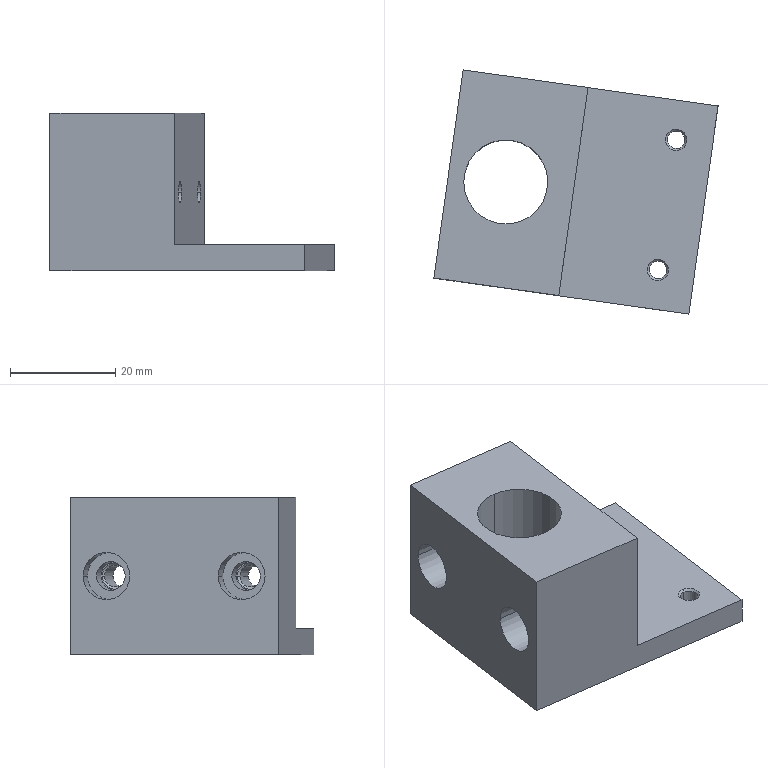Component | SolidWorks | SwitchMount-1 | 1 solid | 38 faces | box 54.1 x 46.44 x 30 mm | volume 26297 mm3 | cylinder 18 | plane 12 | cone 8 | commonest cylinder face diameters 3.3 x4 5.5 x4 4.2 x4 9 x4 16 x2
STEP:
#1=CARTESIAN_POINT('',(-2.788,-8.94,0.7923));
#2=VERTEX_POINT('',#1);
#3=CARTESIAN_POINT('',(-2.806,-9.068,0.7923));
#4=VERTEX_POINT('',#3);
#5=CARTESIAN_POINT('',(-2.797,-9.004,0.7923));
#6=DIRECTION('',(-0.,0.,1.));
#7=DIRECTION('',(-0.1393,-0.9902,0.));
#8=AXIS2_PLACEMENT_3D('',#5,#6,#7);
#9=CIRCLE('',#8,0.06496);
#10=EDGE_CURVE('',#2,#4,#9,.T.);
#11=ORIENTED_EDGE('',*,*,#10,.F.);
#12=CARTESIAN_POINT('',(-2.786,-8.925,0.8071));
#13=VERTEX_POINT('',#12);
#14=CARTESIAN_POINT('',(-2.786,-8.925,0.8071));
#15=DIRECTION('',(0.09852,0.7002,0.7071));
#16=VECTOR('',#15,39.37);
#17=LINE('',#14,#16);
#18=EDGE_CURVE('',#2,#13,#17,.T.);
#19=ORIENTED_EDGE('',*,*,#18,.T.);
#20=CARTESIAN_POINT('',(-2.808,-9.083,0.8071));
#21=VERTEX_POINT('',#20);
#22=CARTESIAN_POINT('',(-2.797,-9.004,0.8071));
#23=DIRECTION('',(-0.,0.,1.));
#24=DIRECTION('',(-0.1393,-0.9902,0.));
#25=AXIS2_PLACEMENT_3D('',#22,#23,#24);
#26=CIRCLE('',#25,0.07972);
#27=EDGE_CURVE('',#13,#21,#26,.T.);
#28=ORIENTED_EDGE('',*,*,#27,.T.);
#29=CARTESIAN_POINT('',(-2.808,-9.083,0.8071));
#30=DIRECTION('',(-0.09852,-0.7002,0.7071));
#31=VECTOR('',#30,39.37);
#32=LINE('',#29,#31);
#33=EDGE_CURVE('',#4,#21,#32,.T.);
#34=ORIENTED_EDGE('',*,*,#33,.F.);
#35=EDGE_LOOP('',(#11,#19,#28,#34));
#36=FACE_OUTER_BOUND('',#35,.T.);
#37=CARTESIAN_POINT('',(-2.797,-9.004,0.8071));
#38=DIRECTION('',(-0.,0.,1.));
#39=DIRECTION('',(-0.1393,-0.9902,0.));
#40=AXIS2_PLACEMENT_3D('',#37,#38,#39);
#41=CONICAL_SURFACE('',#40,0.07972,0.7854);
#42=ADVANCED_FACE('',(#36),#41,.F.);
#43=CARTESIAN_POINT('',(-2.788,-8.94,0.6102));
#44=VERTEX_POINT('',#43);
#45=CARTESIAN_POINT('',(-2.806,-9.068,0.6102));
#46=VERTEX_POINT('',#45);
#47=CARTESIAN_POINT('',(-2.797,-9.004,0.6102));
#48=DIRECTION('',(-0.,0.,1.));
#49=DIRECTION('',(-0.1393,-0.9902,0.));
#50=AXIS2_PLACEMENT_3D('',#47,#48,#49);
#51=CIRCLE('',#50,0.06496);
#52=EDGE_CURVE('',#44,#46,#51,.T.);
#53=ORIENTED_EDGE('',*,*,#52,.F.);
#54=CARTESIAN_POINT('',(-2.788,-8.94,0.8071));
#55=DIRECTION('',(-0.,0.,1.));
#56=VECTOR('',#55,39.37);
#57=LINE('',#54,#56);
#58=EDGE_CURVE('',#44,#2,#57,.T.);
#59=ORIENTED_EDGE('',*,*,#58,.T.);
#60=ORIENTED_EDGE('',*,*,#10,.T.);
#61=CARTESIAN_POINT('',(-2.806,-9.068,0.8071));
#62=DIRECTION('',(-0.,0.,1.));
#63=VECTOR('',#62,39.37);
#64=LINE('',#61,#63);
#65=EDGE_CURVE('',#46,#4,#64,.T.);
#66=ORIENTED_EDGE('',*,*,#65,.F.);
#67=EDGE_LOOP('',(#53,#59,#60,#66));
#68=FACE_OUTER_BOUND('',#67,.T.);
#69=CARTESIAN_POINT('',(-2.797,-9.004,0.8071));
#70=DIRECTION('',(-0.,0.,1.));
#71=DIRECTION('',(-0.1393,-0.9902,0.));
#72=AXIS2_PLACEMENT_3D('',#69,#70,#71);
#73=CYLINDRICAL_SURFACE('',#72,0.06496);
#74=ADVANCED_FACE('',(#68),#73,.F.);
#75=CARTESIAN_POINT('',(-2.651,-7.965,0.7923));
#76=VERTEX_POINT('',#75);
#77=CARTESIAN_POINT('',(-2.669,-8.094,0.7923));
#78=VERTEX_POINT('',#77);
#79=CARTESIAN_POINT('',(-2.66,-8.029,0.7923));
#80=DIRECTION('',(-0.,0.,1.));
#81=DIRECTION('',(-0.1393,-0.9902,0.));
#82=AXIS2_PLACEMENT_3D('',#79,#80,#81);
#83=CIRCLE('',#82,0.06496);
#84=EDGE_CURVE('',#76,#78,#83,.T.);
#85=ORIENTED_EDGE('',*,*,#84,.F.);
#86=CARTESIAN_POINT('',(-2.649,-7.95,0.8071));
#87=VERTEX_POINT('',#86);
#88=CARTESIAN_POINT('',(-2.649,-7.95,0.8071));
#89=DIRECTION('',(0.09852,0.7002,0.7071));
#90=VECTOR('',#89,39.37);
#91=LINE('',#88,#90);
#92=EDGE_CURVE('',#76,#87,#91,.T.);
#93=ORIENTED_EDGE('',*,*,#92,.T.);
#94=CARTESIAN_POINT('',(-2.671,-8.108,0.8071));
#95=VERTEX_POINT('',#94);
#96=CARTESIAN_POINT('',(-2.66,-8.029,0.8071));
#97=DIRECTION('',(-0.,0.,1.));
#98=DIRECTION('',(-0.1393,-0.9902,0.));
#99=AXIS2_PLACEMENT_3D('',#96,#97,#98);
#100=CIRCLE('',#99,0.07972);
#101=EDGE_CURVE('',#87,#95,#100,.T.);
#102=ORIENTED_EDGE('',*,*,#101,.T.);
#103=CARTESIAN_POINT('',(-2.671,-8.108,0.8071));
#104=DIRECTION('',(-0.09852,-0.7002,0.7071));
#105=VECTOR('',#104,39.37);
#106=LINE('',#103,#105);
#107=EDGE_CURVE('',#78,#95,#106,.T.);
#108=ORIENTED_EDGE('',*,*,#107,.F.);
#109=EDGE_LOOP('',(#85,#93,#102,#108));
#110=FACE_OUTER_BOUND('',#109,.T.);
#111=CARTESIAN_POINT('',(-2.66,-8.029,0.8071));
#112=DIRECTION('',(-0.,0.,1.));
#113=DIRECTION('',(-0.1393,-0.9902,0.));
#114=AXIS2_PLACEMENT_3D('',#111,#112,#113);
#115=CONICAL_SURFACE('',#114,0.07972,0.7854);
#116=ADVANCED_FACE('',(#110),#115,.F.);
#117=CARTESIAN_POINT('',(-2.651,-7.965,0.6102));
#118=VERTEX_POINT('',#117);
#119=CARTESIAN_POINT('',(-2.669,-8.094,0.6102));
#120=VERTEX_POINT('',#119);
#121=CARTESIAN_POINT('',(-2.66,-8.029,0.6102));
#122=DIRECTION('',(-0.,0.,1.));
#123=DIRECTION('',(-0.1393,-0.9902,0.));
#124=AXIS2_PLACEMENT_3D('',#121,#122,#123);
#125=CIRCLE('',#124,0.06496);
#126=EDGE_CURVE('',#118,#120,#125,.T.);
#127=ORIENTED_EDGE('',*,*,#126,.F.);
#128=CARTESIAN_POINT('',(-2.651,-7.965,0.8071));
#129=DIRECTION('',(-0.,0.,1.));
#130=VECTOR('',#129,39.37);
#131=LINE('',#128,#130);
#132=EDGE_CURVE('',#118,#76,#131,.T.);
#133=ORIENTED_EDGE('',*,*,#132,.T.);
#134=ORIENTED_EDGE('',*,*,#84,.T.);
#135=CARTESIAN_POINT('',(-2.669,-8.094,0.8071));
#136=DIRECTION('',(-0.,0.,1.));
#137=VECTOR('',#136,39.37);
#138=LINE('',#135,#137);
#139=EDGE_CURVE('',#120,#78,#138,.T.);
#140=ORIENTED_EDGE('',*,*,#139,.F.);
#141=EDGE_LOOP('',(#127,#133,#134,#140));
#142=FACE_OUTER_BOUND('',#141,.T.);
#143=CARTESIAN_POINT('',(-2.66,-8.029,0.8071));
#144=DIRECTION('',(-0.,0.,1.));
#145=DIRECTION('',(-0.1393,-0.9902,0.));
#146=AXIS2_PLACEMENT_3D('',#143,#144,#145);
#147=CYLINDRICAL_SURFACE('',#146,0.06496);
#148=ADVANCED_FACE('',(#142),#147,.F.);
#149=CARTESIAN_POINT('',(-3.981,-8.658,1.791));
#150=VERTEX_POINT('',#149);
#151=CARTESIAN_POINT('',(-3.893,-8.035,1.791));
#152=VERTEX_POINT('',#151);
#153=CARTESIAN_POINT('',(-3.937,-8.346,1.791));
#154=DIRECTION('',(0.,-0.,-1.));
#155=DIRECTION('',(0.1393,0.9902,0.));
#156=AXIS2_PLACEMENT_3D('',#153,#154,#155);
#157=CIRCLE('',#156,0.315);
#158=EDGE_CURVE('',#150,#152,#157,.T.);
#159=ORIENTED_EDGE('',*,*,#158,.F.);
#160=CARTESIAN_POINT('',(-3.981,-8.658,0.6102));
#161=VERTEX_POINT('',#160);
#162=CARTESIAN_POINT('',(-3.981,-8.658,0.6102));
#163=DIRECTION('',(0.,-0.,-1.));
#164=VECTOR('',#163,39.37);
#165=LINE('',#162,#164);
#166=EDGE_CURVE('',#150,#161,#165,.T.);
#167=ORIENTED_EDGE('',*,*,#166,.T.);
#168=CARTESIAN_POINT('',(-3.893,-8.035,0.6102));
#169=VERTEX_POINT('',#168);
#170=CARTESIAN_POINT('',(-3.937,-8.346,0.6102));
#171=DIRECTION('',(0.,-0.,-1.));
#172=DIRECTION('',(0.1393,0.9902,0.));
#173=AXIS2_PLACEMENT_3D('',#170,#171,#172);
#174=CIRCLE('',#173,0.315);
#175=EDGE_CURVE('',#161,#169,#174,.T.);
#176=ORIENTED_EDGE('',*,*,#175,.T.);
#177=CARTESIAN_POINT('',(-3.893,-8.035,0.6102));
#178=DIRECTION('',(0.,-0.,-1.));
#179=VECTOR('',#178,39.37);
#180=LINE('',#177,#179);
#181=EDGE_CURVE('',#152,#169,#180,.T.);
#182=ORIENTED_EDGE('',*,*,#181,.F.);
#183=EDGE_LOOP('',(#159,#167,#176,#182));
#184=FACE_OUTER_BOUND('',#183,.T.);
#185=CARTESIAN_POINT('',(-3.937,-8.346,0.6102));
#186=DIRECTION('',(0.,-0.,-1.));
#187=DIRECTION('',(0.1393,0.9902,0.));
#188=AXIS2_PLACEMENT_3D('',#185,#186,#187);
#189=CYLINDRICAL_SURFACE('',#188,0.315);
#190=ADVANCED_FACE('',(#184),#189,.F.);
#191=CARTESIAN_POINT('',(-4.218,-8.933,1.201));
#192=VERTEX_POINT('',#191);
#193=CARTESIAN_POINT('',(-4.188,-8.719,1.201));
#194=VERTEX_POINT('',#193);
#195=CARTESIAN_POINT('',(-4.203,-8.826,1.201));
#196=DIRECTION('',(0.9902,-0.1393,0.));
#197=DIRECTION('',(0.1393,0.9902,0.));
#198=AXIS2_PLACEMENT_3D('',#195,#196,#197);
#199=CIRCLE('',#198,0.1083);
#200=EDGE_CURVE('',#192,#194,#199,.T.);
#201=ORIENTED_EDGE('',*,*,#200,.F.);
#202=CARTESIAN_POINT('',(-3.984,-8.966,1.201));
#203=VERTEX_POINT('',#202);
#204=CARTESIAN_POINT('',(-4.452,-8.9,1.201));
#205=DIRECTION('',(0.9902,-0.1393,0.));
#206=VECTOR('',#205,39.37);
#207=LINE('',#204,#206);
#208=EDGE_CURVE('',#192,#203,#207,.T.);
#209=ORIENTED_EDGE('',*,*,#208,.T.);
#210=CARTESIAN_POINT('',(-3.954,-8.752,1.201));
#211=VERTEX_POINT('',#210);
#212=CARTESIAN_POINT('',(-3.969,-8.859,1.201));
#213=DIRECTION('',(0.9902,-0.1393,0.));
#214=DIRECTION('',(0.1393,0.9902,0.));
#215=AXIS2_PLACEMENT_3D('',#212,#213,#214);
#216=CIRCLE('',#215,0.1083);
#217=EDGE_CURVE('',#203,#211,#216,.T.);
#218=ORIENTED_EDGE('',*,*,#217,.T.);
#219=CARTESIAN_POINT('',(-4.422,-8.686,1.201));
#220=DIRECTION('',(0.9902,-0.1393,0.));
#221=VECTOR('',#220,39.37);
#222=LINE('',#219,#221);
#223=EDGE_CURVE('',#194,#211,#222,.T.);
#224=ORIENTED_EDGE('',*,*,#223,.F.);
#225=EDGE_LOOP('',(#201,#209,#218,#224));
#226=FACE_OUTER_BOUND('',#225,.T.);
#227=CARTESIAN_POINT('',(-4.437,-8.793,1.201));
#228=DIRECTION('',(0.9902,-0.1393,0.));
#229=DIRECTION('',(0.1393,0.9902,0.));
#230=AXIS2_PLACEMENT_3D('',#227,#228,#229);
#231=CYLINDRICAL_SURFACE('',#230,0.1083);
#232=ADVANCED_FACE('',(#226),#231,.F.);
#233=CARTESIAN_POINT('',(-3.964,-8.943,1.201));
#234=VERTEX_POINT('',#233);
#235=CARTESIAN_POINT('',(-3.941,-8.779,1.201));
#236=VERTEX_POINT('',#235);
#237=CARTESIAN_POINT('',(-3.953,-8.861,1.201));
#238=DIRECTION('',(0.9902,-0.1393,0.));
#239=DIRECTION('',(0.1393,0.9902,0.));
#240=AXIS2_PLACEMENT_3D('',#237,#238,#239);
#241=CIRCLE('',#240,0.08268);
#242=EDGE_CURVE('',#234,#236,#241,.T.);
#243=ORIENTED_EDGE('',*,*,#242,.T.);
#244=CARTESIAN_POINT('',(-3.955,-8.76,1.201));
#245=VERTEX_POINT('',#244);
#246=CARTESIAN_POINT('',(-3.941,-8.779,1.201));
#247=DIRECTION('',(-0.6017,0.7987,0.));
#248=VECTOR('',#247,39.37);
#249=LINE('',#246,#248);
#250=EDGE_CURVE('',#236,#245,#249,.T.);
#251=ORIENTED_EDGE('',*,*,#250,.T.);
#252=CARTESIAN_POINT('',(-3.983,-8.957,1.201));
#253=VERTEX_POINT('',#252);
#254=CARTESIAN_POINT('',(-3.969,-8.859,1.201));
#255=DIRECTION('',(0.9902,-0.1393,0.));
#256=DIRECTION('',(0.1393,0.9902,0.));
#257=AXIS2_PLACEMENT_3D('',#254,#255,#256);
#258=CIRCLE('',#257,0.09941);
#259=EDGE_CURVE('',#253,#245,#258,.T.);
#260=ORIENTED_EDGE('',*,*,#259,.F.);
#261=CARTESIAN_POINT('',(-3.964,-8.943,1.201));
#262=DIRECTION('',(-0.7987,-0.6017,-0.));
#263=VECTOR('',#262,39.37);
#264=LINE('',#261,#263);
#265=EDGE_CURVE('',#234,#253,#264,.T.);
#266=ORIENTED_EDGE('',*,*,#265,.F.);
#267=EDGE_LOOP('',(#243,#251,#260,#266));
#268=FACE_OUTER_BOUND('',#267,.T.);
#269=CARTESIAN_POINT('',(-3.953,-8.861,1.201));
#270=DIRECTION('',(-0.9902,0.1393,-0.));
#271=DIRECTION('',(-0.1393,-0.9902,0.));
#272=AXIS2_PLACEMENT_3D('',#269,#270,#271);
#273=CONICAL_SURFACE('',#272,0.08268,0.7854);
#274=ADVANCED_FACE('',(#268),#273,.F.);
#275=ORIENTED_EDGE('',*,*,#242,.F.);
#276=CARTESIAN_POINT('',(-3.513,-9.006,1.201));
#277=VERTEX_POINT('',#276);
#278=CARTESIAN_POINT('',(-4.449,-8.875,1.201));
#279=DIRECTION('',(0.9902,-0.1393,0.));
#280=VECTOR('',#279,39.37);
#281=LINE('',#278,#280);
#282=EDGE_CURVE('',#234,#277,#281,.T.);
#283=ORIENTED_EDGE('',*,*,#282,.T.);
#284=CARTESIAN_POINT('',(-3.49,-8.843,1.201));
#285=VERTEX_POINT('',#284);
#286=CARTESIAN_POINT('',(-3.502,-8.925,1.201));
#287=DIRECTION('',(0.9902,-0.1393,0.));
#288=DIRECTION('',(0.1393,0.9902,0.));
#289=AXIS2_PLACEMENT_3D('',#286,#287,#288);
#290=CIRCLE('',#289,0.08268);
#291=EDGE_CURVE('',#277,#285,#290,.T.);
#292=ORIENTED_EDGE('',*,*,#291,.T.);
#293=CARTESIAN_POINT('',(-4.426,-8.711,1.201));
#294=DIRECTION('',(0.9902,-0.1393,0.));
#295=VECTOR('',#294,39.37);
#296=LINE('',#293,#295);
#297=EDGE_CURVE('',#236,#285,#296,.T.);
#298=ORIENTED_EDGE('',*,*,#297,.F.);
#299=EDGE_LOOP('',(#275,#283,#292,#298));
#300=FACE_OUTER_BOUND('',#299,.T.);
#301=CARTESIAN_POINT('',(-4.437,-8.793,1.201));
#302=DIRECTION('',(0.9902,-0.1393,0.));
#303=DIRECTION('',(0.1393,0.9902,0.));
#304=AXIS2_PLACEMENT_3D('',#301,#302,#303);
#305=CYLINDRICAL_SURFACE('',#304,0.08268);
#306=ADVANCED_FACE('',(#300),#305,.F.);
#307=CARTESIAN_POINT('',(-4.462,-8.968,1.201));
#308=VERTEX_POINT('',#307);
#309=CARTESIAN_POINT('',(-4.412,-8.617,1.201));
#310=VERTEX_POINT('',#309);
#311=CARTESIAN_POINT('',(-4.437,-8.793,1.201));
#312=DIRECTION('',(0.9902,-0.1393,0.));
#313=DIRECTION('',(0.1393,0.9902,0.));
#314=AXIS2_PLACEMENT_3D('',#311,#312,#313);
#315=CIRCLE('',#314,0.1772);
#316=EDGE_CURVE('',#308,#310,#315,.T.);
#317=ORIENTED_EDGE('',*,*,#316,.F.);
#318=CARTESIAN_POINT('',(-4.228,-9.001,1.201));
#319=VERTEX_POINT('',#318);
#320=CARTESIAN_POINT('',(-4.462,-8.968,1.201));
#321=DIRECTION('',(0.9902,-0.1393,0.));
#322=VECTOR('',#321,39.37);
#323=LINE('',#320,#322);
#324=EDGE_CURVE('',#308,#319,#323,.T.);
#325=ORIENTED_EDGE('',*,*,#324,.T.);
#326=CARTESIAN_POINT('',(-4.179,-8.65,1.201));
#327=VERTEX_POINT('',#326);
#328=CARTESIAN_POINT('',(-4.203,-8.826,1.201));
#329=DIRECTION('',(0.9902,-0.1393,0.));
#330=DIRECTION('',(0.1393,0.9902,0.));
#331=AXIS2_PLACEMENT_3D('',#328,#329,#330);
#332=CIRCLE('',#331,0.1772);
#333=EDGE_CURVE('',#319,#327,#332,.T.);
#334=ORIENTED_EDGE('',*,*,#333,.T.);
#335=CARTESIAN_POINT('',(-4.412,-8.617,1.201));
#336=DIRECTION('',(0.9902,-0.1393,0.));
#337=VECTOR('',#336,39.37);
#338=LINE('',#335,#337);
#339=EDGE_CURVE('',#310,#327,#338,.T.);
#340=ORIENTED_EDGE('',*,*,#339,.F.);
#341=EDGE_LOOP('',(#317,#325,#334,#340));
#342=FACE_OUTER_BOUND('',#341,.T.);
#343=CARTESIAN_POINT('',(-4.437,-8.793,1.201));
#344=DIRECTION('',(0.9902,-0.1393,0.));
#345=DIRECTION('',(0.1393,0.9902,0.));
#346=AXIS2_PLACEMENT_3D('',#343,#344,#345);
#347=CYLINDRICAL_SURFACE('',#346,0.1772);
#348=ADVANCED_FACE('',(#342),#347,.F.);
#349=CARTESIAN_POINT('',(-4.076,-7.919,1.201));
#350=VERTEX_POINT('',#349);
#351=CARTESIAN_POINT('',(-4.046,-7.705,1.201));
#352=VERTEX_POINT('',#351);
#353=CARTESIAN_POINT('',(-4.061,-7.812,1.201));
#354=DIRECTION('',(0.9902,-0.1393,0.));
#355=DIRECTION('',(0.1393,0.9902,0.));
#356=AXIS2_PLACEMENT_3D('',#353,#354,#355);
#357=CIRCLE('',#356,0.1083);
#358=EDGE_CURVE('',#350,#352,#357,.T.);
#359=ORIENTED_EDGE('',*,*,#358,.F.);
#360=CARTESIAN_POINT('',(-3.842,-7.952,1.201));
#361=VERTEX_POINT('',#360);
#362=CARTESIAN_POINT('',(-4.31,-7.887,1.201));
#363=DIRECTION('',(0.9902,-0.1393,0.));
#364=VECTOR('',#363,39.37);
#365=LINE('',#362,#364);
#366=EDGE_CURVE('',#350,#361,#365,.T.);
#367=ORIENTED_EDGE('',*,*,#366,.T.);
#368=CARTESIAN_POINT('',(-3.812,-7.738,1.201));
#369=VERTEX_POINT('',#368);
#370=CARTESIAN_POINT('',(-3.827,-7.845,1.201));
#371=DIRECTION('',(0.9902,-0.1393,0.));
#372=DIRECTION('',(0.1393,0.9902,0.));
#373=AXIS2_PLACEMENT_3D('',#370,#371,#372);
#374=CIRCLE('',#373,0.1083);
#375=EDGE_CURVE('',#361,#369,#374,.T.);
#376=ORIENTED_EDGE('',*,*,#375,.T.);
#377=CARTESIAN_POINT('',(-4.279,-7.672,1.201));
#378=DIRECTION('',(0.9902,-0.1393,0.));
#379=VECTOR('',#378,39.37);
#380=LINE('',#377,#379);
#381=EDGE_CURVE('',#352,#369,#380,.T.);
#382=ORIENTED_EDGE('',*,*,#381,.F.);
#383=EDGE_LOOP('',(#359,#367,#376,#382));
#384=FACE_OUTER_BOUND('',#383,.T.);
#385=CARTESIAN_POINT('',(-4.295,-7.779,1.201));
#386=DIRECTION('',(0.9902,-0.1393,0.));
#387=DIRECTION('',(0.1393,0.9902,0.));
#388=AXIS2_PLACEMENT_3D('',#385,#386,#387);
#389=CYLINDRICAL_SURFACE('',#388,0.1083);
#390=ADVANCED_FACE('',(#384),#389,.F.);
#391=CARTESIAN_POINT('',(-3.822,-7.929,1.201));
#392=VERTEX_POINT('',#391);
#393=CARTESIAN_POINT('',(-3.799,-7.766,1.201));
#394=VERTEX_POINT('',#393);
#395=CARTESIAN_POINT('',(-3.81,-7.847,1.201));
#396=DIRECTION('',(0.9902,-0.1393,0.));
#397=DIRECTION('',(0.1393,0.9902,0.));
#398=AXIS2_PLACEMENT_3D('',#395,#396,#397);
#399=CIRCLE('',#398,0.08268);
#400=EDGE_CURVE('',#392,#394,#399,.T.);
#401=ORIENTED_EDGE('',*,*,#400,.T.);
#402=CARTESIAN_POINT('',(-3.813,-7.747,1.201));
#403=VERTEX_POINT('',#402);
#404=CARTESIAN_POINT('',(-3.799,-7.766,1.201));
#405=DIRECTION('',(-0.6017,0.7987,0.));
#406=VECTOR('',#405,39.37);
#407=LINE('',#404,#406);
#408=EDGE_CURVE('',#394,#403,#407,.T.);
#409=ORIENTED_EDGE('',*,*,#408,.T.);
#410=CARTESIAN_POINT('',(-3.841,-7.944,1.201));
#411=VERTEX_POINT('',#410);
#412=CARTESIAN_POINT('',(-3.827,-7.845,1.201));
#413=DIRECTION('',(0.9902,-0.1393,0.));
#414=DIRECTION('',(0.1393,0.9902,0.));
#415=AXIS2_PLACEMENT_3D('',#412,#413,#414);
#416=CIRCLE('',#415,0.09941);
#417=EDGE_CURVE('',#411,#403,#416,.T.);
#418=ORIENTED_EDGE('',*,*,#417,.F.);
#419=CARTESIAN_POINT('',(-3.822,-7.929,1.201));
#420=DIRECTION('',(-0.7987,-0.6017,-0.));
#421=VECTOR('',#420,39.37);
#422=LINE('',#419,#421);
#423=EDGE_CURVE('',#392,#411,#422,.T.);
#424=ORIENTED_EDGE('',*,*,#423,.F.);
#425=EDGE_LOOP('',(#401,#409,#418,#424));
#426=FACE_OUTER_BOUND('',#425,.T.);
#427=CARTESIAN_POINT('',(-3.81,-7.847,1.201));
#428=DIRECTION('',(-0.9902,0.1393,-0.));
#429=DIRECTION('',(-0.1393,-0.9902,0.));
#430=AXIS2_PLACEMENT_3D('',#427,#428,#429);
#431=CONICAL_SURFACE('',#430,0.08268,0.7854);
#432=ADVANCED_FACE('',(#426),#431,.F.);
#433=ORIENTED_EDGE('',*,*,#400,.F.);
#434=CARTESIAN_POINT('',(-3.37,-7.993,1.201));
#435=VERTEX_POINT('',#434);
#436=CARTESIAN_POINT('',(-4.306,-7.861,1.201));
#437=DIRECTION('',(0.9902,-0.1393,0.));
#438=VECTOR('',#437,39.37);
#439=LINE('',#436,#438);
#440=EDGE_CURVE('',#392,#435,#439,.T.);
#441=ORIENTED_EDGE('',*,*,#440,.T.);
#442=CARTESIAN_POINT('',(-3.347,-7.829,1.201));
#443=VERTEX_POINT('',#442);
#444=CARTESIAN_POINT('',(-3.359,-7.911,1.201));
#445=DIRECTION('',(0.9902,-0.1393,0.));
#446=DIRECTION('',(0.1393,0.9902,0.));
#447=AXIS2_PLACEMENT_3D('',#444,#445,#446);
#448=CIRCLE('',#447,0.08268);
#449=EDGE_CURVE('',#435,#443,#448,.T.);
#450=ORIENTED_EDGE('',*,*,#449,.T.);
#451=CARTESIAN_POINT('',(-4.283,-7.697,1.201));
#452=DIRECTION('',(0.9902,-0.1393,0.));
#453=VECTOR('',#452,39.37);
#454=LINE('',#451,#453);
#455=EDGE_CURVE('',#394,#443,#454,.T.);
#456=ORIENTED_EDGE('',*,*,#455,.F.);
#457=EDGE_LOOP('',(#433,#441,#450,#456));
#458=FACE_OUTER_BOUND('',#457,.T.);
#459=CARTESIAN_POINT('',(-4.295,-7.779,1.201));
#460=DIRECTION('',(0.9902,-0.1393,0.));
#461=DIRECTION('',(0.1393,0.9902,0.));
#462=AXIS2_PLACEMENT_3D('',#459,#460,#461);
#463=CYLINDRICAL_SURFACE('',#462,0.08268);
#464=ADVANCED_FACE('',(#458),#463,.F.);
#465=CARTESIAN_POINT('',(-4.319,-7.955,1.201));
#466=VERTEX_POINT('',#465);
#467=CARTESIAN_POINT('',(-4.27,-7.604,1.201));
#468=VERTEX_POINT('',#467);
#469=CARTESIAN_POINT('',(-4.295,-7.779,1.201));
#470=DIRECTION('',(0.9902,-0.1393,0.));
#471=DIRECTION('',(0.1393,0.9902,0.));
#472=AXIS2_PLACEMENT_3D('',#469,#470,#471);
#473=CIRCLE('',#472,0.1772);
#474=EDGE_CURVE('',#466,#468,#473,.T.);
#475=ORIENTED_EDGE('',*,*,#474,.F.);
#476=CARTESIAN_POINT('',(-4.085,-7.988,1.201));
#477=VERTEX_POINT('',#476);
#478=CARTESIAN_POINT('',(-4.319,-7.955,1.201));
#479=DIRECTION('',(0.9902,-0.1393,0.));
#480=VECTOR('',#479,39.37);
#481=LINE('',#478,#480);
#482=EDGE_CURVE('',#466,#477,#481,.T.);
#483=ORIENTED_EDGE('',*,*,#482,.T.);
#484=CARTESIAN_POINT('',(-4.036,-7.637,1.201));
#485=VERTEX_POINT('',#484);
#486=CARTESIAN_POINT('',(-4.061,-7.812,1.201));
#487=DIRECTION('',(0.9902,-0.1393,0.));
#488=DIRECTION('',(0.1393,0.9902,0.));
#489=AXIS2_PLACEMENT_3D('',#486,#487,#488);
#490=CIRCLE('',#489,0.1772);
#491=EDGE_CURVE('',#477,#485,#490,.T.);
#492=ORIENTED_EDGE('',*,*,#491,.T.);
#493=CARTESIAN_POINT('',(-4.27,-7.604,1.201));
#494=DIRECTION('',(0.9902,-0.1393,0.));
#495=VECTOR('',#494,39.37);
#496=LINE('',#493,#495);
#497=EDGE_CURVE('',#468,#485,#496,.T.);
#498=ORIENTED_EDGE('',*,*,#497,.F.);
#499=EDGE_LOOP('',(#475,#483,#492,#498));
#500=FACE_OUTER_BOUND('',#499,.T.);
#501=CARTESIAN_POINT('',(-4.295,-7.779,1.201));
#502=DIRECTION('',(0.9902,-0.1393,0.));
#503=DIRECTION('',(0.1393,0.9902,0.));
#504=AXIS2_PLACEMENT_3D('',#501,#502,#503);
#505=CYLINDRICAL_SURFACE('',#504,0.1772);
#506=ADVANCED_FACE('',(#500),#505,.F.);
#507=CARTESIAN_POINT('',(-2.565,-9.335,0.8071));
#508=VERTEX_POINT('',#507);
#509=CARTESIAN_POINT('',(-2.346,-7.775,0.8071));
#510=VERTEX_POINT('',#509);
#511=CARTESIAN_POINT('',(-2.565,-9.335,0.8071));
#512=DIRECTION('',(0.1393,0.9902,0.));
#513=VECTOR('',#512,39.37);
#514=LINE('',#511,#513);
#515=EDGE_CURVE('',#508,#510,#514,.T.);
#516=ORIENTED_EDGE('',*,*,#515,.F.);
#517=CARTESIAN_POINT('',(-2.565,-9.335,0.6102));
#518=VERTEX_POINT('',#517);
#519=CARTESIAN_POINT('',(-2.565,-9.335,0.6102));
#520=DIRECTION('',(-0.,0.,1.));
#521=VECTOR('',#520,39.37);
#522=LINE('',#519,#521);
#523=EDGE_CURVE('',#518,#508,#522,.T.);
#524=ORIENTED_EDGE('',*,*,#523,.F.);
#525=CARTESIAN_POINT('',(-2.346,-7.775,0.6102));
#526=VERTEX_POINT('',#525);
#527=CARTESIAN_POINT('',(-2.565,-9.335,0.6102));
#528=DIRECTION('',(0.1393,0.9902,0.));
#529=VECTOR('',#528,39.37);
#530=LINE('',#527,#529);
#531=EDGE_CURVE('',#518,#526,#530,.T.);
#532=ORIENTED_EDGE('',*,*,#531,.T.);
#533=CARTESIAN_POINT('',(-2.346,-7.775,0.6102));
#534=DIRECTION('',(-0.,0.,1.));
#535=VECTOR('',#534,39.37);
#536=LINE('',#533,#535);
#537=EDGE_CURVE('',#526,#510,#536,.T.);
#538=ORIENTED_EDGE('',*,*,#537,.T.);
#539=EDGE_LOOP('',(#516,#524,#532,#538));
#540=FACE_OUTER_BOUND('',#539,.T.);
#541=CARTESIAN_POINT('',(-2.565,-9.335,0.6102));
#542=DIRECTION('',(0.9902,-0.1393,0.));
#543=DIRECTION('',(0.1393,0.9902,0.));
#544=AXIS2_PLACEMENT_3D('',#541,#542,#543);
#545=PLANE('',#544);
#546=ADVANCED_FACE('',(#540),#545,.T.);
#547=CARTESIAN_POINT('',(-3.54,-9.197,0.8071));
#548=VERTEX_POINT('',#547);
#549=CARTESIAN_POINT('',(-3.54,-9.197,1.791));
#550=VERTEX_POINT('',#549);
#551=CARTESIAN_POINT('',(-3.54,-9.197,0.8071));
#552=DIRECTION('',(-0.,0.,1.));
#553=VECTOR('',#552,39.37);
#554=LINE('',#551,#553);
#555=EDGE_CURVE('',#548,#550,#554,.T.);
#556=ORIENTED_EDGE('',*,*,#555,.T.);
#557=CARTESIAN_POINT('',(-4.476,-9.066,1.791));
#558=VERTEX_POINT('',#557);
#559=CARTESIAN_POINT('',(-4.476,-9.066,1.791));
#560=DIRECTION('',(0.9902,-0.1393,0.));
#561=VECTOR('',#560,39.37);
#562=LINE('',#559,#561);
#563=EDGE_CURVE('',#558,#550,#562,.T.);
#564=ORIENTED_EDGE('',*,*,#563,.F.);
#565=CARTESIAN_POINT('',(-4.476,-9.066,0.6102));
#566=VERTEX_POINT('',#565);
#567=CARTESIAN_POINT('',(-4.476,-9.066,0.6102));
#568=DIRECTION('',(-0.,0.,1.));
#569=VECTOR('',#568,39.37);
#570=LINE('',#567,#569);
#571=EDGE_CURVE('',#566,#558,#570,.T.);
#572=ORIENTED_EDGE('',*,*,#571,.F.);
#573=CARTESIAN_POINT('',(-4.476,-9.066,0.6102));
#574=DIRECTION('',(0.9902,-0.1393,0.));
#575=VECTOR('',#574,39.37);
#576=LINE('',#573,#575);
#577=EDGE_CURVE('',#566,#518,#576,.T.);
#578=ORIENTED_EDGE('',*,*,#577,.T.);
#579=ORIENTED_EDGE('',*,*,#523,.T.);
#580=CARTESIAN_POINT('',(-2.565,-9.335,0.8071));
#581=DIRECTION('',(-0.9902,0.1393,0.));
#582=VECTOR('',#581,39.37);
#583=LINE('',#580,#582);
#584=EDGE_CURVE('',#508,#548,#583,.T.);
#585=ORIENTED_EDGE('',*,*,#584,.T.);
#586=EDGE_LOOP('',(#556,#564,#572,#578,#579,#585));
#587=FACE_OUTER_BOUND('',#586,.T.);
#588=CARTESIAN_POINT('',(-4.476,-9.066,0.6102));
#589=DIRECTION('',(-0.1393,-0.9902,0.));
#590=DIRECTION('',(0.,-0.,-1.));
#591=AXIS2_PLACEMENT_3D('',#588,#589,#590);
#592=PLANE('',#591);
#593=ADVANCED_FACE('',(#587),#592,.T.);
#594=CARTESIAN_POINT('',(-4.437,-8.793,1.201));
#595=DIRECTION('',(0.9902,-0.1393,0.));
#596=DIRECTION('',(0.1393,0.9902,0.));
#597=AXIS2_PLACEMENT_3D('',#594,#595,#596);
#598=CIRCLE('',#597,0.1772);
#599=EDGE_CURVE('',#310,#308,#598,.T.);
#600=ORIENTED_EDGE('',*,*,#599,.T.);
#601=ORIENTED_EDGE('',*,*,#316,.T.);
#602=EDGE_LOOP('',(#600,#601));
#603=FACE_BOUND('',#602,.T.);
#604=CARTESIAN_POINT('',(-4.295,-7.779,1.201));
#605=DIRECTION('',(0.9902,-0.1393,0.));
#606=DIRECTION('',(0.1393,0.9902,0.));
#607=AXIS2_PLACEMENT_3D('',#604,#605,#606);
#608=CIRCLE('',#607,0.1772);
#609=EDGE_CURVE('',#468,#466,#608,.T.);
#610=ORIENTED_EDGE('',*,*,#609,.T.);
#611=ORIENTED_EDGE('',*,*,#474,.T.);
#612=EDGE_LOOP('',(#610,#611));
#613=FACE_BOUND('',#612,.T.);
#614=CARTESIAN_POINT('',(-4.256,-7.506,1.791));
#615=VERTEX_POINT('',#614);
#616=CARTESIAN_POINT('',(-4.256,-7.506,1.791));
#617=DIRECTION('',(-0.1393,-0.9902,0.));
#618=VECTOR('',#617,39.37);
#619=LINE('',#616,#618);
#620=EDGE_CURVE('',#615,#558,#619,.T.);
#621=ORIENTED_EDGE('',*,*,#620,.F.);
#622=CARTESIAN_POINT('',(-4.256,-7.506,0.6102));
#623=VERTEX_POINT('',#622);
#624=CARTESIAN_POINT('',(-4.256,-7.506,0.6102));
#625=DIRECTION('',(-0.,0.,1.));
#626=VECTOR('',#625,39.37);
#627=LINE('',#624,#626);
#628=EDGE_CURVE('',#623,#615,#627,.T.);
#629=ORIENTED_EDGE('',*,*,#628,.F.);
#630=CARTESIAN_POINT('',(-4.256,-7.506,0.6102));
#631=DIRECTION('',(-0.1393,-0.9902,0.));
#632=VECTOR('',#631,39.37);
#633=LINE('',#630,#632);
#634=EDGE_CURVE('',#623,#566,#633,.T.);
#635=ORIENTED_EDGE('',*,*,#634,.T.);
#636=ORIENTED_EDGE('',*,*,#571,.T.);
#637=EDGE_LOOP('',(#621,#629,#635,#636));
#638=FACE_OUTER_BOUND('',#637,.T.);
#639=CARTESIAN_POINT('',(-4.256,-7.506,0.6102));
#640=DIRECTION('',(-0.9902,0.1393,-0.));
#641=DIRECTION('',(-0.1393,-0.9902,0.));
#642=AXIS2_PLACEMENT_3D('',#639,#640,#641);
#643=PLANE('',#642);
#644=ADVANCED_FACE('',(#603,#613,#638),#643,.T.);
#645=CARTESIAN_POINT('',(-3.32,-7.638,0.8071));
#646=VERTEX_POINT('',#645);
#647=CARTESIAN_POINT('',(-3.32,-7.638,1.791));
#648=VERTEX_POINT('',#647);
#649=CARTESIAN_POINT('',(-3.32,-7.638,0.8071));
#650=DIRECTION('',(-0.,0.,1.));
#651=VECTOR('',#650,39.37);
#652=LINE('',#649,#651);
#653=EDGE_CURVE('',#646,#648,#652,.T.);
#654=ORIENTED_EDGE('',*,*,#653,.F.);
#655=CARTESIAN_POINT('',(-2.346,-7.775,0.8071));
#656=DIRECTION('',(-0.9902,0.1393,0.));
#657=VECTOR('',#656,39.37);
#658=LINE('',#655,#657);
#659=EDGE_CURVE('',#510,#646,#658,.T.);
#660=ORIENTED_EDGE('',*,*,#659,.F.);
#661=ORIENTED_EDGE('',*,*,#537,.F.);
#662=CARTESIAN_POINT('',(-2.346,-7.775,0.6102));
#663=DIRECTION('',(-0.9902,0.1393,-0.));
#664=VECTOR('',#663,39.37);
#665=LINE('',#662,#664);
#666=EDGE_CURVE('',#526,#623,#665,.T.);
#667=ORIENTED_EDGE('',*,*,#666,.T.);
#668=ORIENTED_EDGE('',*,*,#628,.T.);
#669=CARTESIAN_POINT('',(-2.346,-7.775,1.791));
#670=DIRECTION('',(-0.9902,0.1393,-0.));
#671=VECTOR('',#670,39.37);
#672=LINE('',#669,#671);
#673=EDGE_CURVE('',#648,#615,#672,.T.);
#674=ORIENTED_EDGE('',*,*,#673,.F.);
#675=EDGE_LOOP('',(#654,#660,#661,#667,#668,#674));
#676=FACE_OUTER_BOUND('',#675,.T.);
#677=CARTESIAN_POINT('',(-2.346,-7.775,0.6102));
#678=DIRECTION('',(0.1393,0.9902,0.));
#679=DIRECTION('',(-0.,0.,1.));
#680=AXIS2_PLACEMENT_3D('',#677,#678,#679);
#681=PLANE('',#680);
#682=ADVANCED_FACE('',(#676),#681,.T.);
#683=CARTESIAN_POINT('',(-2.797,-9.004,0.6102));
#684=DIRECTION('',(-0.,0.,1.));
#685=DIRECTION('',(-0.1393,-0.9902,0.));
#686=AXIS2_PLACEMENT_3D('',#683,#684,#685);
#687=CIRCLE('',#686,0.06496);
#688=EDGE_CURVE('',#46,#44,#687,.T.);
#689=ORIENTED_EDGE('',*,*,#688,.T.);
#690=ORIENTED_EDGE('',*,*,#52,.T.);
#691=EDGE_LOOP('',(#689,#690));
#692=FACE_BOUND('',#691,.T.);
#693=CARTESIAN_POINT('',(-2.66,-8.029,0.6102));
#694=DIRECTION('',(-0.,0.,1.));
#695=DIRECTION('',(-0.1393,-0.9902,0.));
#696=AXIS2_PLACEMENT_3D('',#693,#694,#695);
#697=CIRCLE('',#696,0.06496);
#698=EDGE_CURVE('',#120,#118,#697,.T.);
#699=ORIENTED_EDGE('',*,*,#698,.T.);
#700=ORIENTED_EDGE('',*,*,#126,.T.);
#701=EDGE_LOOP('',(#699,#700));
#702=FACE_BOUND('',#701,.T.);
#703=CARTESIAN_POINT('',(-3.937,-8.346,0.6102));
#704=DIRECTION('',(0.,-0.,-1.));
#705=DIRECTION('',(0.1393,0.9902,0.));
#706=AXIS2_PLACEMENT_3D('',#703,#704,#705);
#707=CIRCLE('',#706,0.315);
#708=EDGE_CURVE('',#169,#161,#707,.T.);
#709=ORIENTED_EDGE('',*,*,#708,.F.);
#710=ORIENTED_EDGE('',*,*,#175,.F.);
#711=EDGE_LOOP('',(#709,#710));
#712=FACE_BOUND('',#711,.T.);
#713=ORIENTED_EDGE('',*,*,#531,.F.);
#714=ORIENTED_EDGE('',*,*,#577,.F.);
#715=ORIENTED_EDGE('',*,*,#634,.F.);
#716=ORIENTED_EDGE('',*,*,#666,.F.);
#717=EDGE_LOOP('',(#713,#714,#715,#716));
#718=FACE_OUTER_BOUND('',#717,.T.);
#719=CARTESIAN_POINT('',(-4.366,-8.286,0.6102));
#720=DIRECTION('',(-0.,0.,1.));
#721=DIRECTION('',(-0.1393,-0.9902,0.));
#722=AXIS2_PLACEMENT_3D('',#719,#720,#721);
#723=PLANE('',#722);
#724=ADVANCED_FACE('',(#692,#702,#712,#718),#723,.F.);
#725=CARTESIAN_POINT('',(-3.937,-8.346,1.791));
#726=DIRECTION('',(0.,-0.,-1.));
#727=DIRECTION('',(0.1393,0.9902,0.));
#728=AXIS2_PLACEMENT_3D('',#725,#726,#727);
#729=CIRCLE('',#728,0.315);
#730=EDGE_CURVE('',#152,#150,#729,.T.);
#731=ORIENTED_EDGE('',*,*,#730,.T.);
#732=ORIENTED_EDGE('',*,*,#158,.T.);
#733=EDGE_LOOP('',(#731,#732));
#734=FACE_BOUND('',#733,.T.);
#735=CARTESIAN_POINT('',(-3.54,-9.197,1.791));
#736=DIRECTION('',(0.1393,0.9902,0.));
#737=VECTOR('',#736,39.37);
#738=LINE('',#735,#737);
#739=EDGE_CURVE('',#550,#648,#738,.T.);
#740=ORIENTED_EDGE('',*,*,#739,.T.);
#741=ORIENTED_EDGE('',*,*,#673,.T.);
#742=ORIENTED_EDGE('',*,*,#620,.T.);
#743=ORIENTED_EDGE('',*,*,#563,.T.);
#744=EDGE_LOOP('',(#740,#741,#742,#743));
#745=FACE_OUTER_BOUND('',#744,.T.);
#746=CARTESIAN_POINT('',(-4.366,-8.286,1.791));
#747=DIRECTION('',(-0.,0.,1.));
#748=DIRECTION('',(-0.1393,-0.9902,0.));
#749=AXIS2_PLACEMENT_3D('',#746,#747,#748);
#750=PLANE('',#749);
#751=ADVANCED_FACE('',(#734,#745),#750,.T.);
#752=CARTESIAN_POINT('',(-3.502,-8.925,1.201));
#753=DIRECTION('',(0.9902,-0.1393,0.));
#754=DIRECTION('',(0.1393,0.9902,0.));
#755=AXIS2_PLACEMENT_3D('',#752,#753,#754);
#756=CIRCLE('',#755,0.08268);
#757=EDGE_CURVE('',#285,#277,#756,.T.);
#758=ORIENTED_EDGE('',*,*,#757,.F.);
#759=ORIENTED_EDGE('',*,*,#291,.F.);
#760=EDGE_LOOP('',(#758,#759));
#761=FACE_BOUND('',#760,.T.);
#762=CARTESIAN_POINT('',(-3.359,-7.911,1.201));
#763=DIRECTION('',(0.9902,-0.1393,0.));
#764=DIRECTION('',(0.1393,0.9902,0.));
#765=AXIS2_PLACEMENT_3D('',#762,#763,#764);
#766=CIRCLE('',#765,0.08268);
#767=EDGE_CURVE('',#443,#435,#766,.T.);
#768=ORIENTED_EDGE('',*,*,#767,.F.);
#769=ORIENTED_EDGE('',*,*,#449,.F.);
#770=EDGE_LOOP('',(#768,#769));
#771=FACE_BOUND('',#770,.T.);
#772=ORIENTED_EDGE('',*,*,#653,.T.);
#773=ORIENTED_EDGE('',*,*,#739,.F.);
#774=ORIENTED_EDGE('',*,*,#555,.F.);
#775=CARTESIAN_POINT('',(-3.54,-9.197,0.8071));
#776=DIRECTION('',(0.1393,0.9902,0.));
#777=VECTOR('',#776,39.37);
#778=LINE('',#775,#777);
#779=EDGE_CURVE('',#548,#646,#778,.T.);
#780=ORIENTED_EDGE('',*,*,#779,.T.);
#781=EDGE_LOOP('',(#772,#773,#774,#780));
#782=FACE_OUTER_BOUND('',#781,.T.);
#783=CARTESIAN_POINT('',(-3.54,-9.197,0.8071));
#784=DIRECTION('',(-0.9902,0.1393,-0.));
#785=DIRECTION('',(-0.1393,-0.9902,0.));
#786=AXIS2_PLACEMENT_3D('',#783,#784,#785);
#787=PLANE('',#786);
#788=ADVANCED_FACE('',(#761,#771,#782),#787,.F.);
#789=CARTESIAN_POINT('',(-2.797,-9.004,0.8071));
#790=DIRECTION('',(-0.,0.,1.));
#791=DIRECTION('',(-0.1393,-0.9902,0.));
#792=AXIS2_PLACEMENT_3D('',#789,#790,#791);
#793=CIRCLE('',#792,0.07972);
#794=EDGE_CURVE('',#21,#13,#793,.T.);
#795=ORIENTED_EDGE('',*,*,#794,.F.);
#796=ORIENTED_EDGE('',*,*,#27,.F.);
#797=EDGE_LOOP('',(#795,#796));
#798=FACE_BOUND('',#797,.T.);
#799=CARTESIAN_POINT('',(-2.66,-8.029,0.8071));
#800=DIRECTION('',(-0.,0.,1.));
#801=DIRECTION('',(-0.1393,-0.9902,0.));
#802=AXIS2_PLACEMENT_3D('',#799,#800,#801);
#803=CIRCLE('',#802,0.07972);
#804=EDGE_CURVE('',#95,#87,#803,.T.);
#805=ORIENTED_EDGE('',*,*,#804,.F.);
#806=ORIENTED_EDGE('',*,*,#101,.F.);
#807=EDGE_LOOP('',(#805,#806));
#808=FACE_BOUND('',#807,.T.);
#809=ORIENTED_EDGE('',*,*,#659,.T.);
#810=ORIENTED_EDGE('',*,*,#779,.F.);
#811=ORIENTED_EDGE('',*,*,#584,.F.);
#812=ORIENTED_EDGE('',*,*,#515,.T.);
#813=EDGE_LOOP('',(#809,#810,#811,#812));
#814=FACE_OUTER_BOUND('',#813,.T.);
#815=CARTESIAN_POINT('',(-2.565,-9.335,0.8071));
#816=DIRECTION('',(-0.,0.,-1.));
#817=DIRECTION('',(-0.9902,0.1393,0.));
#818=AXIS2_PLACEMENT_3D('',#815,#816,#817);
#819=PLANE('',#818);
#820=ADVANCED_FACE('',(#798,#808,#814),#819,.F.);
#821=ORIENTED_EDGE('',*,*,#482,.F.);
#822=ORIENTED_EDGE('',*,*,#609,.F.);
#823=ORIENTED_EDGE('',*,*,#497,.T.);
#824=CARTESIAN_POINT('',(-4.061,-7.812,1.201));
#825=DIRECTION('',(0.9902,-0.1393,0.));
#826=DIRECTION('',(0.1393,0.9902,0.));
#827=AXIS2_PLACEMENT_3D('',#824,#825,#826);
#828=CIRCLE('',#827,0.1772);
#829=EDGE_CURVE('',#485,#477,#828,.T.);
#830=ORIENTED_EDGE('',*,*,#829,.T.);
#831=EDGE_LOOP('',(#821,#822,#823,#830));
#832=FACE_OUTER_BOUND('',#831,.T.);
#833=CARTESIAN_POINT('',(-4.295,-7.779,1.201));
#834=DIRECTION('',(0.9902,-0.1393,0.));
#835=DIRECTION('',(0.1393,0.9902,0.));
#836=AXIS2_PLACEMENT_3D('',#833,#834,#835);
#837=CYLINDRICAL_SURFACE('',#836,0.1772);
#838=ADVANCED_FACE('',(#832),#837,.F.);
#839=ORIENTED_EDGE('',*,*,#440,.F.);
#840=CARTESIAN_POINT('',(-3.81,-7.847,1.201));
#841=DIRECTION('',(0.9902,-0.1393,0.));
#842=DIRECTION('',(0.1393,0.9902,0.));
#843=AXIS2_PLACEMENT_3D('',#840,#841,#842);
#844=CIRCLE('',#843,0.08268);
#845=EDGE_CURVE('',#394,#392,#844,.T.);
#846=ORIENTED_EDGE('',*,*,#845,.F.);
#847=ORIENTED_EDGE('',*,*,#455,.T.);
#848=ORIENTED_EDGE('',*,*,#767,.T.);
#849=EDGE_LOOP('',(#839,#846,#847,#848));
#850=FACE_OUTER_BOUND('',#849,.T.);
#851=CARTESIAN_POINT('',(-4.295,-7.779,1.201));
#852=DIRECTION('',(0.9902,-0.1393,0.));
#853=DIRECTION('',(0.1393,0.9902,0.));
#854=AXIS2_PLACEMENT_3D('',#851,#852,#853);
#855=CYLINDRICAL_SURFACE('',#854,0.08268);
#856=ADVANCED_FACE('',(#850),#855,.F.);
#857=ORIENTED_EDGE('',*,*,#408,.F.);
#858=ORIENTED_EDGE('',*,*,#845,.T.);
#859=ORIENTED_EDGE('',*,*,#423,.T.);
#860=CARTESIAN_POINT('',(-3.827,-7.845,1.201));
#861=DIRECTION('',(0.9902,-0.1393,0.));
#862=DIRECTION('',(0.1393,0.9902,0.));
#863=AXIS2_PLACEMENT_3D('',#860,#861,#862);
#864=CIRCLE('',#863,0.09941);
#865=EDGE_CURVE('',#403,#411,#864,.T.);
#866=ORIENTED_EDGE('',*,*,#865,.F.);
#867=EDGE_LOOP('',(#857,#858,#859,#866));
#868=FACE_OUTER_BOUND('',#867,.T.);
#869=CARTESIAN_POINT('',(-3.81,-7.847,1.201));
#870=DIRECTION('',(-0.9902,0.1393,-0.));
#871=DIRECTION('',(-0.1393,-0.9902,0.));
#872=AXIS2_PLACEMENT_3D('',#869,#870,#871);
#873=CONICAL_SURFACE('',#872,0.08268,0.7854);
#874=ADVANCED_FACE('',(#868),#873,.F.);
#875=CARTESIAN_POINT('',(-3.827,-7.845,1.201));
#876=DIRECTION('',(0.9902,-0.1393,0.));
#877=DIRECTION('',(0.1393,0.9902,0.));
#878=AXIS2_PLACEMENT_3D('',#875,#876,#877);
#879=CIRCLE('',#878,0.1083);
#880=EDGE_CURVE('',#369,#361,#879,.T.);
#881=ORIENTED_EDGE('',*,*,#880,.F.);
#882=ORIENTED_EDGE('',*,*,#375,.F.);
#883=EDGE_LOOP('',(#881,#882));
#884=FACE_OUTER_BOUND('',#883,.T.);
#885=ORIENTED_EDGE('',*,*,#417,.T.);
#886=ORIENTED_EDGE('',*,*,#865,.T.);
#887=EDGE_LOOP('',(#885,#886));
#888=FACE_BOUND('',#887,.T.);
#889=CARTESIAN_POINT('',(-3.827,-7.845,1.3));
#890=DIRECTION('',(0.9902,-0.1393,0.));
#891=DIRECTION('',(0.1393,0.9902,0.));
#892=AXIS2_PLACEMENT_3D('',#889,#890,#891);
#893=PLANE('',#892);
#894=ADVANCED_FACE('',(#884,#888),#893,.F.);
#895=ORIENTED_EDGE('',*,*,#366,.F.);
#896=CARTESIAN_POINT('',(-4.061,-7.812,1.201));
#897=DIRECTION('',(0.9902,-0.1393,0.));
#898=DIRECTION('',(0.1393,0.9902,0.));
#899=AXIS2_PLACEMENT_3D('',#896,#897,#898);
#900=CIRCLE('',#899,0.1083);
#901=EDGE_CURVE('',#352,#350,#900,.T.);
#902=ORIENTED_EDGE('',*,*,#901,.F.);
#903=ORIENTED_EDGE('',*,*,#381,.T.);
#904=ORIENTED_EDGE('',*,*,#880,.T.);
#905=EDGE_LOOP('',(#895,#902,#903,#904));
#906=FACE_OUTER_BOUND('',#905,.T.);
#907=CARTESIAN_POINT('',(-4.295,-7.779,1.201));
#908=DIRECTION('',(0.9902,-0.1393,0.));
#909=DIRECTION('',(0.1393,0.9902,0.));
#910=AXIS2_PLACEMENT_3D('',#907,#908,#909);
#911=CYLINDRICAL_SURFACE('',#910,0.1083);
#912=ADVANCED_FACE('',(#906),#911,.F.);
#913=ORIENTED_EDGE('',*,*,#829,.F.);
#914=ORIENTED_EDGE('',*,*,#491,.F.);
#915=EDGE_LOOP('',(#913,#914));
#916=FACE_OUTER_BOUND('',#915,.T.);
#917=ORIENTED_EDGE('',*,*,#901,.T.);
#918=ORIENTED_EDGE('',*,*,#358,.T.);
#919=EDGE_LOOP('',(#917,#918));
#920=FACE_BOUND('',#919,.T.);
#921=CARTESIAN_POINT('',(-4.061,-7.812,1.309));
#922=DIRECTION('',(0.9902,-0.1393,0.));
#923=DIRECTION('',(0.1393,0.9902,0.));
#924=AXIS2_PLACEMENT_3D('',#921,#922,#923);
#925=PLANE('',#924);
#926=ADVANCED_FACE('',(#916,#920),#925,.F.);
#927=ORIENTED_EDGE('',*,*,#324,.F.);
#928=ORIENTED_EDGE('',*,*,#599,.F.);
#929=ORIENTED_EDGE('',*,*,#339,.T.);
#930=CARTESIAN_POINT('',(-4.203,-8.826,1.201));
#931=DIRECTION('',(0.9902,-0.1393,0.));
#932=DIRECTION('',(0.1393,0.9902,0.));
#933=AXIS2_PLACEMENT_3D('',#930,#931,#932);
#934=CIRCLE('',#933,0.1772);
#935=EDGE_CURVE('',#327,#319,#934,.T.);
#936=ORIENTED_EDGE('',*,*,#935,.T.);
#937=EDGE_LOOP('',(#927,#928,#929,#936));
#938=FACE_OUTER_BOUND('',#937,.T.);
#939=CARTESIAN_POINT('',(-4.437,-8.793,1.201));
#940=DIRECTION('',(0.9902,-0.1393,0.));
#941=DIRECTION('',(0.1393,0.9902,0.));
#942=AXIS2_PLACEMENT_3D('',#939,#940,#941);
#943=CYLINDRICAL_SURFACE('',#942,0.1772);
#944=ADVANCED_FACE('',(#938),#943,.F.);
#945=ORIENTED_EDGE('',*,*,#282,.F.);
#946=CARTESIAN_POINT('',(-3.953,-8.861,1.201));
#947=DIRECTION('',(0.9902,-0.1393,0.));
#948=DIRECTION('',(0.1393,0.9902,0.));
#949=AXIS2_PLACEMENT_3D('',#946,#947,#948);
#950=CIRCLE('',#949,0.08268);
#951=EDGE_CURVE('',#236,#234,#950,.T.);
#952=ORIENTED_EDGE('',*,*,#951,.F.);
#953=ORIENTED_EDGE('',*,*,#297,.T.);
#954=ORIENTED_EDGE('',*,*,#757,.T.);
#955=EDGE_LOOP('',(#945,#952,#953,#954));
#956=FACE_OUTER_BOUND('',#955,.T.);
#957=CARTESIAN_POINT('',(-4.437,-8.793,1.201));
#958=DIRECTION('',(0.9902,-0.1393,0.));
#959=DIRECTION('',(0.1393,0.9902,0.));
#960=AXIS2_PLACEMENT_3D('',#957,#958,#959);
#961=CYLINDRICAL_SURFACE('',#960,0.08268);
#962=ADVANCED_FACE('',(#956),#961,.F.);
#963=ORIENTED_EDGE('',*,*,#250,.F.);
#964=ORIENTED_EDGE('',*,*,#951,.T.);
#965=ORIENTED_EDGE('',*,*,#265,.T.);
#966=CARTESIAN_POINT('',(-3.969,-8.859,1.201));
#967=DIRECTION('',(0.9902,-0.1393,0.));
#968=DIRECTION('',(0.1393,0.9902,0.));
#969=AXIS2_PLACEMENT_3D('',#966,#967,#968);
#970=CIRCLE('',#969,0.09941);
#971=EDGE_CURVE('',#245,#253,#970,.T.);
#972=ORIENTED_EDGE('',*,*,#971,.F.);
#973=EDGE_LOOP('',(#963,#964,#965,#972));
#974=FACE_OUTER_BOUND('',#973,.T.);
#975=CARTESIAN_POINT('',(-3.953,-8.861,1.201));
#976=DIRECTION('',(-0.9902,0.1393,-0.));
#977=DIRECTION('',(-0.1393,-0.9902,0.));
#978=AXIS2_PLACEMENT_3D('',#975,#976,#977);
#979=CONICAL_SURFACE('',#978,0.08268,0.7854);
#980=ADVANCED_FACE('',(#974),#979,.F.);
#981=CARTESIAN_POINT('',(-3.969,-8.859,1.201));
#982=DIRECTION('',(0.9902,-0.1393,0.));
#983=DIRECTION('',(0.1393,0.9902,0.));
#984=AXIS2_PLACEMENT_3D('',#981,#982,#983);
#985=CIRCLE('',#984,0.1083);
#986=EDGE_CURVE('',#211,#203,#985,.T.);
#987=ORIENTED_EDGE('',*,*,#986,.F.);
#988=ORIENTED_EDGE('',*,*,#217,.F.);
#989=EDGE_LOOP('',(#987,#988));
#990=FACE_OUTER_BOUND('',#989,.T.);
#991=ORIENTED_EDGE('',*,*,#259,.T.);
#992=ORIENTED_EDGE('',*,*,#971,.T.);
#993=EDGE_LOOP('',(#991,#992));
#994=FACE_BOUND('',#993,.T.);
#995=CARTESIAN_POINT('',(-3.969,-8.859,1.3));
#996=DIRECTION('',(0.9902,-0.1393,0.));
#997=DIRECTION('',(0.1393,0.9902,0.));
#998=AXIS2_PLACEMENT_3D('',#995,#996,#997);
#999=PLANE('',#998);
#1000=ADVANCED_FACE('',(#990,#994),#999,.F.);
#1001=ORIENTED_EDGE('',*,*,#208,.F.);
#1002=CARTESIAN_POINT('',(-4.203,-8.826,1.201));
#1003=DIRECTION('',(0.9902,-0.1393,0.));
#1004=DIRECTION('',(0.1393,0.9902,0.));
#1005=AXIS2_PLACEMENT_3D('',#1002,#1003,#1004);
#1006=CIRCLE('',#1005,0.1083);
#1007=EDGE_CURVE('',#194,#192,#1006,.T.);
#1008=ORIENTED_EDGE('',*,*,#1007,.F.);
#1009=ORIENTED_EDGE('',*,*,#223,.T.);
#1010=ORIENTED_EDGE('',*,*,#986,.T.);
#1011=EDGE_LOOP('',(#1001,#1008,#1009,#1010));
#1012=FACE_OUTER_BOUND('',#1011,.T.);
#1013=CARTESIAN_POINT('',(-4.437,-8.793,1.201));
#1014=DIRECTION('',(0.9902,-0.1393,0.));
#1015=DIRECTION('',(0.1393,0.9902,0.));
#1016=AXIS2_PLACEMENT_3D('',#1013,#1014,#1015);
#1017=CYLINDRICAL_SURFACE('',#1016,0.1083);
#1018=ADVANCED_FACE('',(#1012),#1017,.F.);
#1019=ORIENTED_EDGE('',*,*,#935,.F.);
#1020=ORIENTED_EDGE('',*,*,#333,.F.);
#1021=EDGE_LOOP('',(#1019,#1020));
#1022=FACE_OUTER_BOUND('',#1021,.T.);
#1023=ORIENTED_EDGE('',*,*,#1007,.T.);
#1024=ORIENTED_EDGE('',*,*,#200,.T.);
#1025=EDGE_LOOP('',(#1023,#1024));
#1026=FACE_BOUND('',#1025,.T.);
#1027=CARTESIAN_POINT('',(-4.203,-8.826,1.309));
#1028=DIRECTION('',(0.9902,-0.1393,0.));
#1029=DIRECTION('',(0.1393,0.9902,0.));
#1030=AXIS2_PLACEMENT_3D('',#1027,#1028,#1029);
#1031=PLANE('',#1030);
#1032=ADVANCED_FACE('',(#1022,#1026),#1031,.F.);
#1033=ORIENTED_EDGE('',*,*,#166,.F.);
#1034=ORIENTED_EDGE('',*,*,#730,.F.);
#1035=ORIENTED_EDGE('',*,*,#181,.T.);
#1036=ORIENTED_EDGE('',*,*,#708,.T.);
#1037=EDGE_LOOP('',(#1033,#1034,#1035,#1036));
#1038=FACE_OUTER_BOUND('',#1037,.T.);
#1039=CARTESIAN_POINT('',(-3.937,-8.346,0.6102));
#1040=DIRECTION('',(0.,-0.,-1.));
#1041=DIRECTION('',(0.1393,0.9902,0.));
#1042=AXIS2_PLACEMENT_3D('',#1039,#1040,#1041);
#1043=CYLINDRICAL_SURFACE('',#1042,0.315);
#1044=ADVANCED_FACE('',(#1038),#1043,.F.);
#1045=ORIENTED_EDGE('',*,*,#132,.F.);
#1046=ORIENTED_EDGE('',*,*,#698,.F.);
#1047=ORIENTED_EDGE('',*,*,#139,.T.);
#1048=CARTESIAN_POINT('',(-2.66,-8.029,0.7923));
#1049=DIRECTION('',(-0.,0.,1.));
#1050=DIRECTION('',(-0.1393,-0.9902,0.));
#1051=AXIS2_PLACEMENT_3D('',#1048,#1049,#1050);
#1052=CIRCLE('',#1051,0.06496);
#1053=EDGE_CURVE('',#78,#76,#1052,.T.);
#1054=ORIENTED_EDGE('',*,*,#1053,.T.);
#1055=EDGE_LOOP('',(#1045,#1046,#1047,#1054));
#1056=FACE_OUTER_BOUND('',#1055,.T.);
#1057=CARTESIAN_POINT('',(-2.66,-8.029,0.8071));
#1058=DIRECTION('',(-0.,0.,1.));
#1059=DIRECTION('',(-0.1393,-0.9902,0.));
#1060=AXIS2_PLACEMENT_3D('',#1057,#1058,#1059);
#1061=CYLINDRICAL_SURFACE('',#1060,0.06496);
#1062=ADVANCED_FACE('',(#1056),#1061,.F.);
#1063=ORIENTED_EDGE('',*,*,#92,.F.);
#1064=ORIENTED_EDGE('',*,*,#1053,.F.);
#1065=ORIENTED_EDGE('',*,*,#107,.T.);
#1066=ORIENTED_EDGE('',*,*,#804,.T.);
#1067=EDGE_LOOP('',(#1063,#1064,#1065,#1066));
#1068=FACE_OUTER_BOUND('',#1067,.T.);
#1069=CARTESIAN_POINT('',(-2.66,-8.029,0.8071));
#1070=DIRECTION('',(-0.,0.,1.));
#1071=DIRECTION('',(-0.1393,-0.9902,0.));
#1072=AXIS2_PLACEMENT_3D('',#1069,#1070,#1071);
#1073=CONICAL_SURFACE('',#1072,0.07972,0.7854);
#1074=ADVANCED_FACE('',(#1068),#1073,.F.);
#1075=ORIENTED_EDGE('',*,*,#58,.F.);
#1076=ORIENTED_EDGE('',*,*,#688,.F.);
#1077=ORIENTED_EDGE('',*,*,#65,.T.);
#1078=CARTESIAN_POINT('',(-2.797,-9.004,0.7923));
#1079=DIRECTION('',(-0.,0.,1.));
#1080=DIRECTION('',(-0.1393,-0.9902,0.));
#1081=AXIS2_PLACEMENT_3D('',#1078,#1079,#1080);
#1082=CIRCLE('',#1081,0.06496);
#1083=EDGE_CURVE('',#4,#2,#1082,.T.);
#1084=ORIENTED_EDGE('',*,*,#1083,.T.);
#1085=EDGE_LOOP('',(#1075,#1076,#1077,#1084));
#1086=FACE_OUTER_BOUND('',#1085,.T.);
#1087=CARTESIAN_POINT('',(-2.797,-9.004,0.8071));
#1088=DIRECTION('',(-0.,0.,1.));
#1089=DIRECTION('',(-0.1393,-0.9902,0.));
#1090=AXIS2_PLACEMENT_3D('',#1087,#1088,#1089);
#1091=CYLINDRICAL_SURFACE('',#1090,0.06496);
#1092=ADVANCED_FACE('',(#1086),#1091,.F.);
#1093=ORIENTED_EDGE('',*,*,#18,.F.);
#1094=ORIENTED_EDGE('',*,*,#1083,.F.);
#1095=ORIENTED_EDGE('',*,*,#33,.T.);
#1096=ORIENTED_EDGE('',*,*,#794,.T.);
#1097=EDGE_LOOP('',(#1093,#1094,#1095,#1096));
#1098=FACE_OUTER_BOUND('',#1097,.T.);
#1099=CARTESIAN_POINT('',(-2.797,-9.004,0.8071));
#1100=DIRECTION('',(-0.,0.,1.));
#1101=DIRECTION('',(-0.1393,-0.9902,0.));
#1102=AXIS2_PLACEMENT_3D('',#1099,#1100,#1101);
#1103=CONICAL_SURFACE('',#1102,0.07972,0.7854);
#1104=ADVANCED_FACE('',(#1098),#1103,.F.);
#1105=CLOSED_SHELL('',(#42,#74,#116,#148,#190,#232,#274,#306,#348,#390,#432,#464,#506,#546,#593,#644,#682,#724,#751,#788,#820,#838,#856,#874,#894,#912,#926,#944,#962,#980,#1000,#1018,#1032,#1044,#1062,#1074,#1092,#1104));
#1106=MANIFOLD_SOLID_BREP('',#1105);
#1107=CARTESIAN_POINT('',(0.,0.,0.));
#1108=DIRECTION('',(0.,0.,1.));
#1109=DIRECTION('',(1.,0.,0.));
#1110=AXIS2_PLACEMENT_3D('',#1107,#1108,#1109);
#1111=(LENGTH_UNIT()NAMED_UNIT(*)SI_UNIT($,.METRE.));
#1112=LENGTH_MEASURE_WITH_UNIT(LENGTH_MEASURE(0.0254),#1111);
#1113=DIMENSIONAL_EXPONENTS(1.,0.,0.,0.,0.,0.,0.);
#1114=(CONVERSION_BASED_UNIT('',#1112)LENGTH_UNIT()NAMED_UNIT(#1113));
#1115=UNCERTAINTY_MEASURE_WITH_UNIT(LENGTH_MEASURE(0.00001),#1114,'','');
#1116=(NAMED_UNIT(*)PLANE_ANGLE_UNIT()SI_UNIT($,.RADIAN.));
#1117=(NAMED_UNIT(*)SI_UNIT($,.STERADIAN.)SOLID_ANGLE_UNIT());
#1118=(GEOMETRIC_REPRESENTATION_CONTEXT(3)GLOBAL_UNCERTAINTY_ASSIGNED_CONTEXT((#1115))GLOBAL_UNIT_ASSIGNED_CONTEXT((#1114,#1116,#1117))REPRESENTATION_CONTEXT('',''));
#1119=ADVANCED_BREP_SHAPE_REPRESENTATION('',(#1106,#1110),#1118);
#1120=COLOUR_RGB('',0.7922,0.8196,0.9333);
#1121=FILL_AREA_STYLE_COLOUR('',#1120);
#1122=FILL_AREA_STYLE('',(#1121));
#1123=SURFACE_STYLE_FILL_AREA(#1122);
#1124=SURFACE_SIDE_STYLE('',(#1123));
#1125=SURFACE_STYLE_USAGE(.BOTH.,#1124);
#1126=PRESENTATION_STYLE_ASSIGNMENT((#1125));
#1127=STYLED_ITEM('',(#1126),#1106);
#1128=PRESENTATION_LAYER_ASSIGNMENT('','',(#1127));
#1129=(LENGTH_UNIT()NAMED_UNIT(*)SI_UNIT($,.METRE.));
#1130=LENGTH_MEASURE_WITH_UNIT(LENGTH_MEASURE(0.0254),#1129);
#1131=DIMENSIONAL_EXPONENTS(1.,0.,0.,0.,0.,0.,0.);
#1132=(CONVERSION_BASED_UNIT('',#1130)LENGTH_UNIT()NAMED_UNIT(#1131));
#1133=UNCERTAINTY_MEASURE_WITH_UNIT(LENGTH_MEASURE(0.00001),#1132,'','');
#1134=(NAMED_UNIT(*)PLANE_ANGLE_UNIT()SI_UNIT($,.RADIAN.));
#1135=(NAMED_UNIT(*)SI_UNIT($,.STERADIAN.)SOLID_ANGLE_UNIT());
#1136=(GEOMETRIC_REPRESENTATION_CONTEXT(3)GLOBAL_UNCERTAINTY_ASSIGNED_CONTEXT((#1133))GLOBAL_UNIT_ASSIGNED_CONTEXT((#1132,#1134,#1135))REPRESENTATION_CONTEXT('',''));
#1137=MECHANICAL_DESIGN_GEOMETRIC_PRESENTATION_REPRESENTATION('',(#1127),#1136);